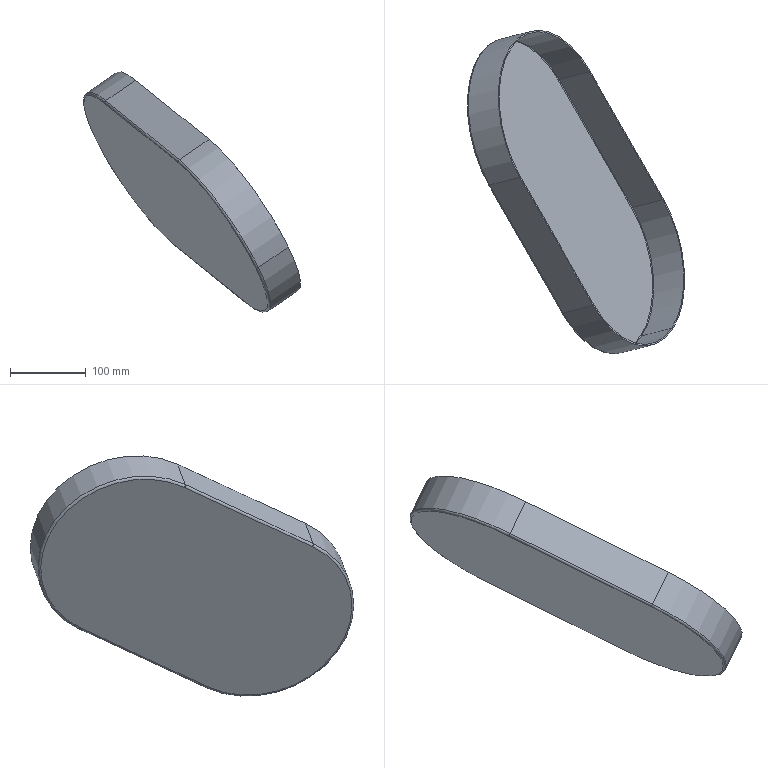Component | SolidWorks | CrusherGearCover-1 | 1 solid | 26 faces | box 287.16 x 427.76 x 317.89 mm | volume 327104 mm3 | cylinder 10 | plane 10 | torus 6 | commonest cylinder face diameters 254 x3 250 x3 2 x2 6 x2
STEP:
#1=COLOUR_RGB('',0.7922,0.8196,0.9333);
#2=FILL_AREA_STYLE_COLOUR('',#1);
#3=FILL_AREA_STYLE('',(#2));
#4=SURFACE_STYLE_FILL_AREA(#3);
#5=SURFACE_SIDE_STYLE('',(#4));
#6=SURFACE_STYLE_USAGE(.BOTH.,#5);
#7=PRESENTATION_STYLE_ASSIGNMENT((#6));
#8=CARTESIAN_POINT('',(-17.886,-16.774,-15.753));
#9=VERTEX_POINT('',#8);
#10=CARTESIAN_POINT('',(-13.854,-17.995,-21.223));
#11=VERTEX_POINT('',#10);
#12=CARTESIAN_POINT('',(-16.107,-14.065,-19.404));
#13=DIRECTION('',(0.8088,0.2094,0.5495));
#14=DIRECTION('',(0.4616,-0.8051,-0.3726));
#15=AXIS2_PLACEMENT_3D('',#12,#13,#14);
#16=CIRCLE('',#15,4.882);
#17=EDGE_CURVE('',#9,#11,#16,.T.);
#18=ORIENTED_EDGE('',*,*,#17,.T.);
#19=CARTESIAN_POINT('',(-13.704,-18.065,-21.202));
#20=VERTEX_POINT('',#19);
#21=CARTESIAN_POINT('',(-13.758,-17.97,-21.158));
#22=DIRECTION('',(-0.3643,-0.555,0.7478));
#23=DIRECTION('',(0.,-0.803,-0.596));
#24=AXIS2_PLACEMENT_3D('',#21,#22,#23);
#25=CIRCLE('',#24,0.1181);
#26=EDGE_CURVE('',#11,#20,#25,.T.);
#27=ORIENTED_EDGE('',*,*,#26,.T.);
#28=CARTESIAN_POINT('',(-17.833,-16.815,-15.6));
#29=VERTEX_POINT('',#28);
#30=CARTESIAN_POINT('',(-16.012,-14.04,-19.339));
#31=DIRECTION('',(0.8088,0.2094,0.5495));
#32=DIRECTION('',(0.4616,-0.8051,-0.3726));
#33=AXIS2_PLACEMENT_3D('',#30,#31,#32);
#34=CIRCLE('',#33,5.);
#35=EDGE_CURVE('',#29,#20,#34,.T.);
#36=ORIENTED_EDGE('',*,*,#35,.F.);
#37=CARTESIAN_POINT('',(-17.79,-16.75,-15.688));
#38=DIRECTION('',(-0.4616,0.8051,0.3726));
#39=DIRECTION('',(-0.3643,-0.555,0.7478));
#40=AXIS2_PLACEMENT_3D('',#37,#38,#39);
#41=CIRCLE('',#40,0.1181);
#42=EDGE_CURVE('',#9,#29,#41,.T.);
#43=ORIENTED_EDGE('',*,*,#42,.F.);
#44=EDGE_LOOP('',(#18,#27,#36,#43));
#45=FACE_OUTER_BOUND('',#44,.T.);
#46=CARTESIAN_POINT('',(-16.012,-14.04,-19.339));
#47=DIRECTION('',(0.8088,0.2094,0.5495));
#48=DIRECTION('',(0.4616,-0.8051,-0.3726));
#49=AXIS2_PLACEMENT_3D('',#46,#47,#48);
#50=TOROIDAL_SURFACE('',#49,4.882,0.1181);
#51=ADVANCED_FACE('',(#45),#50,.T.);
#52=ORIENTED_EDGE('',*,*,#35,.T.);
#53=CARTESIAN_POINT('',(-12.144,-17.661,-20.142));
#54=VERTEX_POINT('',#53);
#55=CARTESIAN_POINT('',(-13.736,-18.074,-21.224));
#56=DIRECTION('',(0.8088,0.2094,0.5495));
#57=VECTOR('',#56,39.37);
#58=LINE('',#55,#57);
#59=EDGE_CURVE('',#20,#54,#58,.T.);
#60=ORIENTED_EDGE('',*,*,#59,.T.);
#61=CARTESIAN_POINT('',(-16.273,-16.411,-14.54));
#62=VERTEX_POINT('',#61);
#63=CARTESIAN_POINT('',(-14.451,-13.636,-18.279));
#64=DIRECTION('',(0.8088,0.2094,0.5495));
#65=DIRECTION('',(0.4616,-0.8051,-0.3726));
#66=AXIS2_PLACEMENT_3D('',#63,#64,#65);
#67=CIRCLE('',#66,5.);
#68=EDGE_CURVE('',#62,#54,#67,.T.);
#69=ORIENTED_EDGE('',*,*,#68,.F.);
#70=CARTESIAN_POINT('',(-17.865,-16.824,-15.621));
#71=DIRECTION('',(0.8088,0.2094,0.5495));
#72=VECTOR('',#71,39.37);
#73=LINE('',#70,#72);
#74=EDGE_CURVE('',#29,#62,#73,.T.);
#75=ORIENTED_EDGE('',*,*,#74,.F.);
#76=EDGE_LOOP('',(#52,#60,#69,#75));
#77=FACE_OUTER_BOUND('',#76,.T.);
#78=CARTESIAN_POINT('',(-16.044,-14.048,-19.361));
#79=DIRECTION('',(0.8088,0.2094,0.5495));
#80=DIRECTION('',(0.4616,-0.8051,-0.3726));
#81=AXIS2_PLACEMENT_3D('',#78,#79,#80);
#82=CYLINDRICAL_SURFACE('',#81,5.);
#83=ADVANCED_FACE('',(#77),#82,.T.);
#84=CARTESIAN_POINT('',(-13.79,-17.979,-21.18));
#85=VERTEX_POINT('',#84);
#86=CARTESIAN_POINT('',(-14.265,-11.339,-23.011));
#87=VERTEX_POINT('',#86);
#88=CARTESIAN_POINT('',(-16.044,-14.048,-19.361));
#89=DIRECTION('',(0.8088,0.2094,0.5495));
#90=DIRECTION('',(-0.3643,-0.555,0.7478));
#91=AXIS2_PLACEMENT_3D('',#88,#89,#90);
#92=CIRCLE('',#91,4.882);
#93=EDGE_CURVE('',#85,#87,#92,.T.);
#94=ORIENTED_EDGE('',*,*,#93,.F.);
#95=CARTESIAN_POINT('',(-13.74,-18.002,-21.173));
#96=VERTEX_POINT('',#95);
#97=CARTESIAN_POINT('',(-13.758,-17.97,-21.158));
#98=DIRECTION('',(-0.3643,-0.555,0.7478));
#99=DIRECTION('',(0.,-0.803,-0.596));
#100=AXIS2_PLACEMENT_3D('',#97,#98,#99);
#101=CIRCLE('',#100,0.03937);
#102=EDGE_CURVE('',#85,#96,#101,.T.);
#103=ORIENTED_EDGE('',*,*,#102,.T.);
#104=CARTESIAN_POINT('',(-14.219,-11.309,-23.019));
#105=VERTEX_POINT('',#104);
#106=CARTESIAN_POINT('',(-16.012,-14.04,-19.339));
#107=DIRECTION('',(0.8088,0.2094,0.5495));
#108=DIRECTION('',(-0.3643,-0.555,0.7478));
#109=AXIS2_PLACEMENT_3D('',#106,#107,#108);
#110=CIRCLE('',#109,4.921);
#111=EDGE_CURVE('',#96,#105,#110,.T.);
#112=ORIENTED_EDGE('',*,*,#111,.T.);
#113=CARTESIAN_POINT('',(-14.233,-11.331,-22.99));
#114=DIRECTION('',(0.4616,-0.8051,-0.3726));
#115=DIRECTION('',(0.8088,0.2094,0.5495));
#116=AXIS2_PLACEMENT_3D('',#113,#114,#115);
#117=CIRCLE('',#116,0.03937);
#118=EDGE_CURVE('',#87,#105,#117,.T.);
#119=ORIENTED_EDGE('',*,*,#118,.F.);
#120=EDGE_LOOP('',(#94,#103,#112,#119));
#121=FACE_OUTER_BOUND('',#120,.T.);
#122=CARTESIAN_POINT('',(-16.012,-14.04,-19.339));
#123=DIRECTION('',(0.8088,0.2094,0.5495));
#124=DIRECTION('',(0.4616,-0.8051,-0.3726));
#125=AXIS2_PLACEMENT_3D('',#122,#123,#124);
#126=TOROIDAL_SURFACE('',#125,4.882,0.03937);
#127=ADVANCED_FACE('',(#121),#126,.F.);
#128=ORIENTED_EDGE('',*,*,#111,.F.);
#129=CARTESIAN_POINT('',(-12.18,-17.598,-20.113));
#130=VERTEX_POINT('',#129);
#131=CARTESIAN_POINT('',(-13.772,-18.01,-21.194));
#132=DIRECTION('',(0.8088,0.2094,0.5495));
#133=VECTOR('',#132,39.37);
#134=LINE('',#131,#133);
#135=EDGE_CURVE('',#96,#130,#134,.T.);
#136=ORIENTED_EDGE('',*,*,#135,.T.);
#137=CARTESIAN_POINT('',(-12.658,-10.905,-21.959));
#138=VERTEX_POINT('',#137);
#139=CARTESIAN_POINT('',(-14.451,-13.636,-18.279));
#140=DIRECTION('',(0.8088,0.2094,0.5495));
#141=DIRECTION('',(-0.3643,-0.555,0.7478));
#142=AXIS2_PLACEMENT_3D('',#139,#140,#141);
#143=CIRCLE('',#142,4.921);
#144=EDGE_CURVE('',#130,#138,#143,.T.);
#145=ORIENTED_EDGE('',*,*,#144,.T.);
#146=CARTESIAN_POINT('',(-14.251,-11.317,-23.041));
#147=DIRECTION('',(0.8088,0.2094,0.5495));
#148=VECTOR('',#147,39.37);
#149=LINE('',#146,#148);
#150=EDGE_CURVE('',#105,#138,#149,.T.);
#151=ORIENTED_EDGE('',*,*,#150,.F.);
#152=EDGE_LOOP('',(#128,#136,#145,#151));
#153=FACE_OUTER_BOUND('',#152,.T.);
#154=CARTESIAN_POINT('',(-16.044,-14.048,-19.361));
#155=DIRECTION('',(0.8088,0.2094,0.5495));
#156=DIRECTION('',(0.4616,-0.8051,-0.3726));
#157=AXIS2_PLACEMENT_3D('',#154,#155,#156);
#158=CYLINDRICAL_SURFACE('',#157,4.921);
#159=ADVANCED_FACE('',(#153),#158,.F.);
#160=CARTESIAN_POINT('',(-16.446,-4.205,-18.937));
#161=VERTEX_POINT('',#160);
#162=CARTESIAN_POINT('',(-16.475,-4.249,-18.878));
#163=VERTEX_POINT('',#162);
#164=CARTESIAN_POINT('',(-16.475,-4.249,-18.878));
#165=DIRECTION('',(-0.3643,-0.555,0.7478));
#166=VECTOR('',#165,39.37);
#167=LINE('',#164,#166);
#168=EDGE_CURVE('',#161,#163,#167,.T.);
#169=ORIENTED_EDGE('',*,*,#168,.F.);
#170=CARTESIAN_POINT('',(-20.089,-9.755,-11.459));
#171=VERTEX_POINT('',#170);
#172=CARTESIAN_POINT('',(-18.268,-6.98,-15.198));
#173=DIRECTION('',(0.8088,0.2094,0.5495));
#174=DIRECTION('',(0.4616,-0.8051,-0.3726));
#175=AXIS2_PLACEMENT_3D('',#172,#173,#174);
#176=CIRCLE('',#175,5.);
#177=EDGE_CURVE('',#161,#171,#176,.T.);
#178=ORIENTED_EDGE('',*,*,#177,.T.);
#179=CARTESIAN_POINT('',(-20.061,-9.712,-11.518));
#180=VERTEX_POINT('',#179);
#181=CARTESIAN_POINT('',(-20.061,-9.712,-11.518));
#182=DIRECTION('',(0.3643,0.555,-0.7478));
#183=VECTOR('',#182,39.37);
#184=LINE('',#181,#183);
#185=EDGE_CURVE('',#171,#180,#184,.T.);
#186=ORIENTED_EDGE('',*,*,#185,.T.);
#187=CARTESIAN_POINT('',(-18.268,-6.98,-15.198));
#188=DIRECTION('',(0.8088,0.2094,0.5495));
#189=DIRECTION('',(0.3643,0.555,-0.7478));
#190=AXIS2_PLACEMENT_3D('',#187,#188,#189);
#191=CIRCLE('',#190,4.921);
#192=EDGE_CURVE('',#163,#180,#191,.T.);
#193=ORIENTED_EDGE('',*,*,#192,.F.);
#194=EDGE_LOOP('',(#169,#178,#186,#193));
#195=FACE_OUTER_BOUND('',#194,.T.);
#196=CARTESIAN_POINT('',(-18.268,-6.98,-15.198));
#197=DIRECTION('',(-0.8088,-0.2094,-0.5495));
#198=DIRECTION('',(-0.4616,0.8051,0.3726));
#199=AXIS2_PLACEMENT_3D('',#196,#197,#198);
#200=PLANE('',#199);
#201=ADVANCED_FACE('',(#195),#200,.F.);
#202=ORIENTED_EDGE('',*,*,#185,.F.);
#203=CARTESIAN_POINT('',(-20.089,-9.755,-11.459));
#204=DIRECTION('',(0.4616,-0.8051,-0.3726));
#205=VECTOR('',#204,39.37);
#206=LINE('',#203,#205);
#207=EDGE_CURVE('',#171,#62,#206,.T.);
#208=ORIENTED_EDGE('',*,*,#207,.T.);
#209=CARTESIAN_POINT('',(-16.244,-16.368,-14.599));
#210=VERTEX_POINT('',#209);
#211=CARTESIAN_POINT('',(-16.244,-16.368,-14.599));
#212=DIRECTION('',(0.3643,0.555,-0.7478));
#213=VECTOR('',#212,39.37);
#214=LINE('',#211,#213);
#215=EDGE_CURVE('',#62,#210,#214,.T.);
#216=ORIENTED_EDGE('',*,*,#215,.T.);
#217=CARTESIAN_POINT('',(-20.061,-9.712,-11.518));
#218=DIRECTION('',(0.4616,-0.8051,-0.3726));
#219=VECTOR('',#218,39.37);
#220=LINE('',#217,#219);
#221=EDGE_CURVE('',#180,#210,#220,.T.);
#222=ORIENTED_EDGE('',*,*,#221,.F.);
#223=EDGE_LOOP('',(#202,#208,#216,#222));
#224=FACE_OUTER_BOUND('',#223,.T.);
#225=CARTESIAN_POINT('',(-20.061,-9.712,-11.518));
#226=DIRECTION('',(0.8088,0.2094,0.5495));
#227=DIRECTION('',(0.4616,-0.8051,-0.3726));
#228=AXIS2_PLACEMENT_3D('',#225,#226,#227);
#229=PLANE('',#228);
#230=ADVANCED_FACE('',(#224),#229,.T.);
#231=ORIENTED_EDGE('',*,*,#215,.F.);
#232=ORIENTED_EDGE('',*,*,#68,.T.);
#233=CARTESIAN_POINT('',(-12.63,-10.861,-22.018));
#234=VERTEX_POINT('',#233);
#235=CARTESIAN_POINT('',(-14.451,-13.636,-18.279));
#236=DIRECTION('',(0.8088,0.2094,0.5495));
#237=DIRECTION('',(0.4616,-0.8051,-0.3726));
#238=AXIS2_PLACEMENT_3D('',#235,#236,#237);
#239=CIRCLE('',#238,5.);
#240=EDGE_CURVE('',#54,#234,#239,.T.);
#241=ORIENTED_EDGE('',*,*,#240,.T.);
#242=CARTESIAN_POINT('',(-12.658,-10.905,-21.959));
#243=DIRECTION('',(-0.3643,-0.555,0.7478));
#244=VECTOR('',#243,39.37);
#245=LINE('',#242,#244);
#246=EDGE_CURVE('',#234,#138,#245,.T.);
#247=ORIENTED_EDGE('',*,*,#246,.T.);
#248=ORIENTED_EDGE('',*,*,#144,.F.);
#249=CARTESIAN_POINT('',(-14.451,-13.636,-18.279));
#250=DIRECTION('',(0.8088,0.2094,0.5495));
#251=DIRECTION('',(-0.3643,-0.555,0.7478));
#252=AXIS2_PLACEMENT_3D('',#249,#250,#251);
#253=CIRCLE('',#252,4.921);
#254=EDGE_CURVE('',#210,#130,#253,.T.);
#255=ORIENTED_EDGE('',*,*,#254,.F.);
#256=EDGE_LOOP('',(#231,#232,#241,#247,#248,#255));
#257=FACE_OUTER_BOUND('',#256,.T.);
#258=CARTESIAN_POINT('',(-14.451,-13.636,-18.279));
#259=DIRECTION('',(-0.8088,-0.2094,-0.5495));
#260=DIRECTION('',(-0.4616,0.8051,0.3726));
#261=AXIS2_PLACEMENT_3D('',#258,#259,#260);
#262=PLANE('',#261);
#263=ADVANCED_FACE('',(#257),#262,.F.);
#264=CARTESIAN_POINT('',(-12.63,-10.861,-22.018));
#265=DIRECTION('',(-0.4616,0.8051,0.3726));
#266=VECTOR('',#265,39.37);
#267=LINE('',#264,#266);
#268=EDGE_CURVE('',#234,#161,#267,.T.);
#269=ORIENTED_EDGE('',*,*,#268,.T.);
#270=ORIENTED_EDGE('',*,*,#168,.T.);
#271=CARTESIAN_POINT('',(-12.658,-10.905,-21.959));
#272=DIRECTION('',(-0.4616,0.8051,0.3726));
#273=VECTOR('',#272,39.37);
#274=LINE('',#271,#273);
#275=EDGE_CURVE('',#138,#163,#274,.T.);
#276=ORIENTED_EDGE('',*,*,#275,.F.);
#277=ORIENTED_EDGE('',*,*,#246,.F.);
#278=EDGE_LOOP('',(#269,#270,#276,#277));
#279=FACE_OUTER_BOUND('',#278,.T.);
#280=CARTESIAN_POINT('',(-12.658,-10.905,-21.959));
#281=DIRECTION('',(0.8088,0.2094,0.5495));
#282=DIRECTION('',(-0.4616,0.8051,0.3726));
#283=AXIS2_PLACEMENT_3D('',#280,#281,#282);
#284=PLANE('',#283);
#285=ADVANCED_FACE('',(#279),#284,.T.);
#286=ORIENTED_EDGE('',*,*,#135,.F.);
#287=CARTESIAN_POINT('',(-17.805,-16.772,-15.659));
#288=VERTEX_POINT('',#287);
#289=CARTESIAN_POINT('',(-16.012,-14.04,-19.339));
#290=DIRECTION('',(0.8088,0.2094,0.5495));
#291=DIRECTION('',(-0.3643,-0.555,0.7478));
#292=AXIS2_PLACEMENT_3D('',#289,#290,#291);
#293=CIRCLE('',#292,4.921);
#294=EDGE_CURVE('',#288,#96,#293,.T.);
#295=ORIENTED_EDGE('',*,*,#294,.F.);
#296=CARTESIAN_POINT('',(-17.837,-16.78,-15.68));
#297=DIRECTION('',(0.8088,0.2094,0.5495));
#298=VECTOR('',#297,39.37);
#299=LINE('',#296,#298);
#300=EDGE_CURVE('',#288,#210,#299,.T.);
#301=ORIENTED_EDGE('',*,*,#300,.T.);
#302=ORIENTED_EDGE('',*,*,#254,.T.);
#303=EDGE_LOOP('',(#286,#295,#301,#302));
#304=FACE_OUTER_BOUND('',#303,.T.);
#305=CARTESIAN_POINT('',(-16.044,-14.048,-19.361));
#306=DIRECTION('',(0.8088,0.2094,0.5495));
#307=DIRECTION('',(0.4616,-0.8051,-0.3726));
#308=AXIS2_PLACEMENT_3D('',#305,#306,#307);
#309=CYLINDRICAL_SURFACE('',#308,4.921);
#310=ADVANCED_FACE('',(#304),#309,.F.);
#311=ORIENTED_EDGE('',*,*,#102,.F.);
#312=CARTESIAN_POINT('',(-17.822,-16.758,-15.71));
#313=VERTEX_POINT('',#312);
#314=CARTESIAN_POINT('',(-16.044,-14.048,-19.361));
#315=DIRECTION('',(0.8088,0.2094,0.5495));
#316=DIRECTION('',(-0.3643,-0.555,0.7478));
#317=AXIS2_PLACEMENT_3D('',#314,#315,#316);
#318=CIRCLE('',#317,4.882);
#319=EDGE_CURVE('',#313,#85,#318,.T.);
#320=ORIENTED_EDGE('',*,*,#319,.F.);
#321=CARTESIAN_POINT('',(-17.79,-16.75,-15.688));
#322=DIRECTION('',(-0.4616,0.8051,0.3726));
#323=DIRECTION('',(0.8088,0.2094,0.5495));
#324=AXIS2_PLACEMENT_3D('',#321,#322,#323);
#325=CIRCLE('',#324,0.03937);
#326=EDGE_CURVE('',#313,#288,#325,.T.);
#327=ORIENTED_EDGE('',*,*,#326,.T.);
#328=ORIENTED_EDGE('',*,*,#294,.T.);
#329=EDGE_LOOP('',(#311,#320,#327,#328));
#330=FACE_OUTER_BOUND('',#329,.T.);
#331=CARTESIAN_POINT('',(-16.012,-14.04,-19.339));
#332=DIRECTION('',(0.8088,0.2094,0.5495));
#333=DIRECTION('',(0.4616,-0.8051,-0.3726));
#334=AXIS2_PLACEMENT_3D('',#331,#332,#333);
#335=TOROIDAL_SURFACE('',#334,4.882,0.03937);
#336=ADVANCED_FACE('',(#330),#335,.F.);
#337=ORIENTED_EDGE('',*,*,#221,.T.);
#338=ORIENTED_EDGE('',*,*,#300,.F.);
#339=CARTESIAN_POINT('',(-21.621,-10.116,-12.578));
#340=VERTEX_POINT('',#339);
#341=CARTESIAN_POINT('',(-21.621,-10.116,-12.578));
#342=DIRECTION('',(0.4616,-0.8051,-0.3726));
#343=VECTOR('',#342,39.37);
#344=LINE('',#341,#343);
#345=EDGE_CURVE('',#340,#288,#344,.T.);
#346=ORIENTED_EDGE('',*,*,#345,.F.);
#347=CARTESIAN_POINT('',(-21.653,-10.124,-12.6));
#348=DIRECTION('',(0.8088,0.2094,0.5495));
#349=VECTOR('',#348,39.37);
#350=LINE('',#347,#349);
#351=EDGE_CURVE('',#340,#180,#350,.T.);
#352=ORIENTED_EDGE('',*,*,#351,.T.);
#353=EDGE_LOOP('',(#337,#338,#346,#352));
#354=FACE_OUTER_BOUND('',#353,.T.);
#355=CARTESIAN_POINT('',(-21.653,-10.124,-12.6));
#356=DIRECTION('',(0.3643,0.555,-0.7478));
#357=DIRECTION('',(0.8088,0.2094,0.5495));
#358=AXIS2_PLACEMENT_3D('',#355,#356,#357);
#359=PLANE('',#358);
#360=ADVANCED_FACE('',(#354),#359,.T.);
#361=ORIENTED_EDGE('',*,*,#345,.T.);
#362=ORIENTED_EDGE('',*,*,#326,.F.);
#363=CARTESIAN_POINT('',(-21.638,-10.102,-12.629));
#364=VERTEX_POINT('',#363);
#365=CARTESIAN_POINT('',(-21.638,-10.102,-12.629));
#366=DIRECTION('',(0.4616,-0.8051,-0.3726));
#367=VECTOR('',#366,39.37);
#368=LINE('',#365,#367);
#369=EDGE_CURVE('',#364,#313,#368,.T.);
#370=ORIENTED_EDGE('',*,*,#369,.F.);
#371=CARTESIAN_POINT('',(-21.607,-10.094,-12.607));
#372=DIRECTION('',(-0.4616,0.8051,0.3726));
#373=DIRECTION('',(0.8088,0.2094,0.5495));
#374=AXIS2_PLACEMENT_3D('',#371,#372,#373);
#375=CIRCLE('',#374,0.03937);
#376=EDGE_CURVE('',#364,#340,#375,.T.);
#377=ORIENTED_EDGE('',*,*,#376,.T.);
#378=EDGE_LOOP('',(#361,#362,#370,#377));
#379=FACE_OUTER_BOUND('',#378,.T.);
#380=CARTESIAN_POINT('',(-21.607,-10.094,-12.607));
#381=DIRECTION('',(0.4616,-0.8051,-0.3726));
#382=DIRECTION('',(-0.8088,-0.2094,-0.5495));
#383=AXIS2_PLACEMENT_3D('',#380,#381,#382);
#384=CYLINDRICAL_SURFACE('',#383,0.03937);
#385=ADVANCED_FACE('',(#379),#384,.F.);
#386=ORIENTED_EDGE('',*,*,#192,.T.);
#387=ORIENTED_EDGE('',*,*,#351,.F.);
#388=CARTESIAN_POINT('',(-18.035,-4.653,-19.938));
#389=VERTEX_POINT('',#388);
#390=CARTESIAN_POINT('',(-19.828,-7.384,-16.258));
#391=DIRECTION('',(0.8088,0.2094,0.5495));
#392=DIRECTION('',(0.3643,0.555,-0.7478));
#393=AXIS2_PLACEMENT_3D('',#390,#391,#392);
#394=CIRCLE('',#393,4.921);
#395=EDGE_CURVE('',#389,#340,#394,.T.);
#396=ORIENTED_EDGE('',*,*,#395,.F.);
#397=CARTESIAN_POINT('',(-18.067,-4.661,-19.96));
#398=DIRECTION('',(0.8088,0.2094,0.5495));
#399=VECTOR('',#398,39.37);
#400=LINE('',#397,#399);
#401=EDGE_CURVE('',#389,#163,#400,.T.);
#402=ORIENTED_EDGE('',*,*,#401,.T.);
#403=EDGE_LOOP('',(#386,#387,#396,#402));
#404=FACE_OUTER_BOUND('',#403,.T.);
#405=CARTESIAN_POINT('',(-19.86,-7.393,-16.28));
#406=DIRECTION('',(0.8088,0.2094,0.5495));
#407=DIRECTION('',(0.4616,-0.8051,-0.3726));
#408=AXIS2_PLACEMENT_3D('',#405,#406,#407);
#409=CYLINDRICAL_SURFACE('',#408,4.921);
#410=ADVANCED_FACE('',(#404),#409,.F.);
#411=ORIENTED_EDGE('',*,*,#395,.T.);
#412=ORIENTED_EDGE('',*,*,#376,.F.);
#413=CARTESIAN_POINT('',(-18.081,-4.683,-19.931));
#414=VERTEX_POINT('',#413);
#415=CARTESIAN_POINT('',(-19.86,-7.393,-16.28));
#416=DIRECTION('',(0.8088,0.2094,0.5495));
#417=DIRECTION('',(0.3643,0.555,-0.7478));
#418=AXIS2_PLACEMENT_3D('',#415,#416,#417);
#419=CIRCLE('',#418,4.882);
#420=EDGE_CURVE('',#414,#364,#419,.T.);
#421=ORIENTED_EDGE('',*,*,#420,.F.);
#422=CARTESIAN_POINT('',(-18.049,-4.675,-19.909));
#423=DIRECTION('',(0.4616,-0.8051,-0.3726));
#424=DIRECTION('',(0.8088,0.2094,0.5495));
#425=AXIS2_PLACEMENT_3D('',#422,#423,#424);
#426=CIRCLE('',#425,0.03937);
#427=EDGE_CURVE('',#414,#389,#426,.T.);
#428=ORIENTED_EDGE('',*,*,#427,.T.);
#429=EDGE_LOOP('',(#411,#412,#421,#428));
#430=FACE_OUTER_BOUND('',#429,.T.);
#431=CARTESIAN_POINT('',(-19.828,-7.384,-16.258));
#432=DIRECTION('',(0.8088,0.2094,0.5495));
#433=DIRECTION('',(0.4616,-0.8051,-0.3726));
#434=AXIS2_PLACEMENT_3D('',#431,#432,#433);
#435=TOROIDAL_SURFACE('',#434,4.882,0.03937);
#436=ADVANCED_FACE('',(#430),#435,.F.);
#437=ORIENTED_EDGE('',*,*,#275,.T.);
#438=ORIENTED_EDGE('',*,*,#401,.F.);
#439=CARTESIAN_POINT('',(-14.219,-11.309,-23.019));
#440=DIRECTION('',(-0.4616,0.8051,0.3726));
#441=VECTOR('',#440,39.37);
#442=LINE('',#439,#441);
#443=EDGE_CURVE('',#105,#389,#442,.T.);
#444=ORIENTED_EDGE('',*,*,#443,.F.);
#445=ORIENTED_EDGE('',*,*,#150,.T.);
#446=EDGE_LOOP('',(#437,#438,#444,#445));
#447=FACE_OUTER_BOUND('',#446,.T.);
#448=CARTESIAN_POINT('',(-14.251,-11.317,-23.041));
#449=DIRECTION('',(-0.3643,-0.555,0.7478));
#450=DIRECTION('',(-0.8088,-0.2094,-0.5495));
#451=AXIS2_PLACEMENT_3D('',#448,#449,#450);
#452=PLANE('',#451);
#453=ADVANCED_FACE('',(#447),#452,.T.);
#454=ORIENTED_EDGE('',*,*,#443,.T.);
#455=ORIENTED_EDGE('',*,*,#427,.F.);
#456=CARTESIAN_POINT('',(-14.265,-11.339,-23.011));
#457=DIRECTION('',(-0.4616,0.8051,0.3726));
#458=VECTOR('',#457,39.37);
#459=LINE('',#456,#458);
#460=EDGE_CURVE('',#87,#414,#459,.T.);
#461=ORIENTED_EDGE('',*,*,#460,.F.);
#462=ORIENTED_EDGE('',*,*,#118,.T.);
#463=EDGE_LOOP('',(#454,#455,#461,#462));
#464=FACE_OUTER_BOUND('',#463,.T.);
#465=CARTESIAN_POINT('',(-14.233,-11.331,-22.99));
#466=DIRECTION('',(-0.4616,0.8051,0.3726));
#467=DIRECTION('',(0.8088,0.2094,0.5495));
#468=AXIS2_PLACEMENT_3D('',#465,#466,#467);
#469=CYLINDRICAL_SURFACE('',#468,0.03937);
#470=ADVANCED_FACE('',(#464),#469,.F.);
#471=ORIENTED_EDGE('',*,*,#59,.F.);
#472=CARTESIAN_POINT('',(-14.19,-11.265,-23.078));
#473=VERTEX_POINT('',#472);
#474=CARTESIAN_POINT('',(-16.012,-14.04,-19.339));
#475=DIRECTION('',(0.8088,0.2094,0.5495));
#476=DIRECTION('',(0.4616,-0.8051,-0.3726));
#477=AXIS2_PLACEMENT_3D('',#474,#475,#476);
#478=CIRCLE('',#477,5.);
#479=EDGE_CURVE('',#20,#473,#478,.T.);
#480=ORIENTED_EDGE('',*,*,#479,.T.);
#481=CARTESIAN_POINT('',(-14.222,-11.273,-23.1));
#482=DIRECTION('',(0.8088,0.2094,0.5495));
#483=VECTOR('',#482,39.37);
#484=LINE('',#481,#483);
#485=EDGE_CURVE('',#473,#234,#484,.T.);
#486=ORIENTED_EDGE('',*,*,#485,.T.);
#487=ORIENTED_EDGE('',*,*,#240,.F.);
#488=EDGE_LOOP('',(#471,#480,#486,#487));
#489=FACE_OUTER_BOUND('',#488,.T.);
#490=CARTESIAN_POINT('',(-16.044,-14.048,-19.361));
#491=DIRECTION('',(0.8088,0.2094,0.5495));
#492=DIRECTION('',(0.4616,-0.8051,-0.3726));
#493=AXIS2_PLACEMENT_3D('',#490,#491,#492);
#494=CYLINDRICAL_SURFACE('',#493,5.);
#495=ADVANCED_FACE('',(#489),#494,.T.);
#496=ORIENTED_EDGE('',*,*,#26,.F.);
#497=CARTESIAN_POINT('',(-14.329,-11.355,-23.055));
#498=VERTEX_POINT('',#497);
#499=CARTESIAN_POINT('',(-16.107,-14.065,-19.404));
#500=DIRECTION('',(0.8088,0.2094,0.5495));
#501=DIRECTION('',(0.4616,-0.8051,-0.3726));
#502=AXIS2_PLACEMENT_3D('',#499,#500,#501);
#503=CIRCLE('',#502,4.882);
#504=EDGE_CURVE('',#11,#498,#503,.T.);
#505=ORIENTED_EDGE('',*,*,#504,.T.);
#506=CARTESIAN_POINT('',(-14.233,-11.331,-22.99));
#507=DIRECTION('',(0.4616,-0.8051,-0.3726));
#508=DIRECTION('',(0.8088,0.2094,0.5495));
#509=AXIS2_PLACEMENT_3D('',#506,#507,#508);
#510=CIRCLE('',#509,0.1181);
#511=EDGE_CURVE('',#498,#473,#510,.T.);
#512=ORIENTED_EDGE('',*,*,#511,.T.);
#513=ORIENTED_EDGE('',*,*,#479,.F.);
#514=EDGE_LOOP('',(#496,#505,#512,#513));
#515=FACE_OUTER_BOUND('',#514,.T.);
#516=CARTESIAN_POINT('',(-16.012,-14.04,-19.339));
#517=DIRECTION('',(0.8088,0.2094,0.5495));
#518=DIRECTION('',(0.4616,-0.8051,-0.3726));
#519=AXIS2_PLACEMENT_3D('',#516,#517,#518);
#520=TOROIDAL_SURFACE('',#519,4.882,0.1181);
#521=ADVANCED_FACE('',(#515),#520,.T.);
#522=ORIENTED_EDGE('',*,*,#207,.F.);
#523=CARTESIAN_POINT('',(-21.65,-10.159,-12.519));
#524=VERTEX_POINT('',#523);
#525=CARTESIAN_POINT('',(-21.681,-10.168,-12.541));
#526=DIRECTION('',(0.8088,0.2094,0.5495));
#527=VECTOR('',#526,39.37);
#528=LINE('',#525,#527);
#529=EDGE_CURVE('',#524,#171,#528,.T.);
#530=ORIENTED_EDGE('',*,*,#529,.F.);
#531=CARTESIAN_POINT('',(-21.65,-10.159,-12.519));
#532=DIRECTION('',(0.4616,-0.8051,-0.3726));
#533=VECTOR('',#532,39.37);
#534=LINE('',#531,#533);
#535=EDGE_CURVE('',#524,#29,#534,.T.);
#536=ORIENTED_EDGE('',*,*,#535,.T.);
#537=ORIENTED_EDGE('',*,*,#74,.T.);
#538=EDGE_LOOP('',(#522,#530,#536,#537));
#539=FACE_OUTER_BOUND('',#538,.T.);
#540=CARTESIAN_POINT('',(-21.681,-10.168,-12.541));
#541=DIRECTION('',(0.3643,0.555,-0.7478));
#542=DIRECTION('',(0.8088,0.2094,0.5495));
#543=AXIS2_PLACEMENT_3D('',#540,#541,#542);
#544=PLANE('',#543);
#545=ADVANCED_FACE('',(#539),#544,.F.);
#546=ORIENTED_EDGE('',*,*,#535,.F.);
#547=CARTESIAN_POINT('',(-21.702,-10.119,-12.672));
#548=VERTEX_POINT('',#547);
#549=CARTESIAN_POINT('',(-21.607,-10.094,-12.607));
#550=DIRECTION('',(-0.4616,0.8051,0.3726));
#551=DIRECTION('',(-0.8088,-0.2094,-0.5495));
#552=AXIS2_PLACEMENT_3D('',#549,#550,#551);
#553=CIRCLE('',#552,0.1181);
#554=EDGE_CURVE('',#548,#524,#553,.T.);
#555=ORIENTED_EDGE('',*,*,#554,.F.);
#556=CARTESIAN_POINT('',(-19.794,-13.447,-14.213));
#557=DIRECTION('',(0.4616,-0.8051,-0.3726));
#558=VECTOR('',#557,39.37);
#559=LINE('',#556,#558);
#560=EDGE_CURVE('',#548,#9,#559,.T.);
#561=ORIENTED_EDGE('',*,*,#560,.T.);
#562=ORIENTED_EDGE('',*,*,#42,.T.);
#563=EDGE_LOOP('',(#546,#555,#561,#562));
#564=FACE_OUTER_BOUND('',#563,.T.);
#565=CARTESIAN_POINT('',(-21.607,-10.094,-12.607));
#566=DIRECTION('',(0.4616,-0.8051,-0.3726));
#567=DIRECTION('',(-0.8088,-0.2094,-0.5495));
#568=AXIS2_PLACEMENT_3D('',#565,#566,#567);
#569=CYLINDRICAL_SURFACE('',#568,0.1181);
#570=ADVANCED_FACE('',(#564),#569,.T.);
#571=ORIENTED_EDGE('',*,*,#177,.F.);
#572=CARTESIAN_POINT('',(-18.006,-4.609,-19.997));
#573=VERTEX_POINT('',#572);
#574=CARTESIAN_POINT('',(-18.038,-4.617,-20.019));
#575=DIRECTION('',(0.8088,0.2094,0.5495));
#576=VECTOR('',#575,39.37);
#577=LINE('',#574,#576);
#578=EDGE_CURVE('',#573,#161,#577,.T.);
#579=ORIENTED_EDGE('',*,*,#578,.F.);
#580=CARTESIAN_POINT('',(-19.828,-7.384,-16.258));
#581=DIRECTION('',(0.8088,0.2094,0.5495));
#582=DIRECTION('',(0.4616,-0.8051,-0.3726));
#583=AXIS2_PLACEMENT_3D('',#580,#581,#582);
#584=CIRCLE('',#583,5.);
#585=EDGE_CURVE('',#573,#524,#584,.T.);
#586=ORIENTED_EDGE('',*,*,#585,.T.);
#587=ORIENTED_EDGE('',*,*,#529,.T.);
#588=EDGE_LOOP('',(#571,#579,#586,#587));
#589=FACE_OUTER_BOUND('',#588,.T.);
#590=CARTESIAN_POINT('',(-19.86,-7.393,-16.28));
#591=DIRECTION('',(0.8088,0.2094,0.5495));
#592=DIRECTION('',(0.4616,-0.8051,-0.3726));
#593=AXIS2_PLACEMENT_3D('',#590,#591,#592);
#594=CYLINDRICAL_SURFACE('',#593,5.);
#595=ADVANCED_FACE('',(#589),#594,.T.);
#596=ORIENTED_EDGE('',*,*,#585,.F.);
#597=CARTESIAN_POINT('',(-18.145,-4.7,-19.974));
#598=VERTEX_POINT('',#597);
#599=CARTESIAN_POINT('',(-18.049,-4.675,-19.909));
#600=DIRECTION('',(0.4616,-0.8051,-0.3726));
#601=DIRECTION('',(0.3643,0.555,-0.7478));
#602=AXIS2_PLACEMENT_3D('',#599,#600,#601);
#603=CIRCLE('',#602,0.1181);
#604=EDGE_CURVE('',#598,#573,#603,.T.);
#605=ORIENTED_EDGE('',*,*,#604,.F.);
#606=CARTESIAN_POINT('',(-19.923,-7.409,-16.323));
#607=DIRECTION('',(0.8088,0.2094,0.5495));
#608=DIRECTION('',(0.4616,-0.8051,-0.3726));
#609=AXIS2_PLACEMENT_3D('',#606,#607,#608);
#610=CIRCLE('',#609,4.882);
#611=EDGE_CURVE('',#598,#548,#610,.T.);
#612=ORIENTED_EDGE('',*,*,#611,.T.);
#613=ORIENTED_EDGE('',*,*,#554,.T.);
#614=EDGE_LOOP('',(#596,#605,#612,#613));
#615=FACE_OUTER_BOUND('',#614,.T.);
#616=CARTESIAN_POINT('',(-19.828,-7.384,-16.258));
#617=DIRECTION('',(0.8088,0.2094,0.5495));
#618=DIRECTION('',(0.4616,-0.8051,-0.3726));
#619=AXIS2_PLACEMENT_3D('',#616,#617,#618);
#620=TOROIDAL_SURFACE('',#619,4.882,0.1181);
#621=ADVANCED_FACE('',(#615),#620,.T.);
#622=ORIENTED_EDGE('',*,*,#268,.F.);
#623=ORIENTED_EDGE('',*,*,#485,.F.);
#624=CARTESIAN_POINT('',(-14.19,-11.265,-23.078));
#625=DIRECTION('',(-0.4616,0.8051,0.3726));
#626=VECTOR('',#625,39.37);
#627=LINE('',#624,#626);
#628=EDGE_CURVE('',#473,#573,#627,.T.);
#629=ORIENTED_EDGE('',*,*,#628,.T.);
#630=ORIENTED_EDGE('',*,*,#578,.T.);
#631=EDGE_LOOP('',(#622,#623,#629,#630));
#632=FACE_OUTER_BOUND('',#631,.T.);
#633=CARTESIAN_POINT('',(-14.222,-11.273,-23.1));
#634=DIRECTION('',(-0.3643,-0.555,0.7478));
#635=DIRECTION('',(-0.8088,-0.2094,-0.5495));
#636=AXIS2_PLACEMENT_3D('',#633,#634,#635);
#637=PLANE('',#636);
#638=ADVANCED_FACE('',(#632),#637,.F.);
#639=ORIENTED_EDGE('',*,*,#628,.F.);
#640=ORIENTED_EDGE('',*,*,#511,.F.);
#641=CARTESIAN_POINT('',(-14.329,-11.355,-23.055));
#642=DIRECTION('',(-0.4616,0.8051,0.3726));
#643=VECTOR('',#642,39.37);
#644=LINE('',#641,#643);
#645=EDGE_CURVE('',#498,#598,#644,.T.);
#646=ORIENTED_EDGE('',*,*,#645,.T.);
#647=ORIENTED_EDGE('',*,*,#604,.T.);
#648=EDGE_LOOP('',(#639,#640,#646,#647));
#649=FACE_OUTER_BOUND('',#648,.T.);
#650=CARTESIAN_POINT('',(-14.233,-11.331,-22.99));
#651=DIRECTION('',(-0.4616,0.8051,0.3726));
#652=DIRECTION('',(0.8088,0.2094,0.5495));
#653=AXIS2_PLACEMENT_3D('',#650,#651,#652);
#654=CYLINDRICAL_SURFACE('',#653,0.1181);
#655=ADVANCED_FACE('',(#649),#654,.T.);
#656=ORIENTED_EDGE('',*,*,#319,.T.);
#657=ORIENTED_EDGE('',*,*,#93,.T.);
#658=ORIENTED_EDGE('',*,*,#460,.T.);
#659=ORIENTED_EDGE('',*,*,#420,.T.);
#660=ORIENTED_EDGE('',*,*,#369,.T.);
#661=EDGE_LOOP('',(#656,#657,#658,#659,#660));
#662=FACE_OUTER_BOUND('',#661,.T.);
#663=CARTESIAN_POINT('',(-19.86,-7.393,-16.28));
#664=DIRECTION('',(0.8088,0.2094,0.5495));
#665=DIRECTION('',(0.4616,-0.8051,-0.3726));
#666=AXIS2_PLACEMENT_3D('',#663,#664,#665);
#667=PLANE('',#666);
#668=ADVANCED_FACE('',(#662),#667,.T.);
#669=ORIENTED_EDGE('',*,*,#645,.F.);
#670=ORIENTED_EDGE('',*,*,#504,.F.);
#671=ORIENTED_EDGE('',*,*,#17,.F.);
#672=ORIENTED_EDGE('',*,*,#560,.F.);
#673=ORIENTED_EDGE('',*,*,#611,.F.);
#674=EDGE_LOOP('',(#669,#670,#671,#672,#673));
#675=FACE_OUTER_BOUND('',#674,.T.);
#676=CARTESIAN_POINT('',(-19.923,-7.409,-16.323));
#677=DIRECTION('',(0.8088,0.2094,0.5495));
#678=DIRECTION('',(0.4616,-0.8051,-0.3726));
#679=AXIS2_PLACEMENT_3D('',#676,#677,#678);
#680=PLANE('',#679);
#681=ADVANCED_FACE('',(#675),#680,.F.);
#682=CLOSED_SHELL('',(#51,#83,#127,#159,#201,#230,#263,#285,#310,#336,#360,#385,#410,#436,#453,#470,#495,#521,#545,#570,#595,#621,#638,#655,#668,#681));
#683=MANIFOLD_SOLID_BREP('',#682);
#684=STYLED_ITEM('',(#7),#683);
#685=(LENGTH_UNIT()NAMED_UNIT(*)SI_UNIT($,.METRE.));
#686=LENGTH_MEASURE_WITH_UNIT(LENGTH_MEASURE(0.0254),#685);
#687=DIMENSIONAL_EXPONENTS(1.,0.,0.,0.,0.,0.,0.);
#688=(CONVERSION_BASED_UNIT('',#686)LENGTH_UNIT()NAMED_UNIT(#687));
#689=UNCERTAINTY_MEASURE_WITH_UNIT(LENGTH_MEASURE(0.00001),#688,'','');
#690=(NAMED_UNIT(*)PLANE_ANGLE_UNIT()SI_UNIT($,.RADIAN.));
#691=(NAMED_UNIT(*)SI_UNIT($,.STERADIAN.)SOLID_ANGLE_UNIT());
#692=(GEOMETRIC_REPRESENTATION_CONTEXT(3)GLOBAL_UNCERTAINTY_ASSIGNED_CONTEXT((#689))GLOBAL_UNIT_ASSIGNED_CONTEXT((#688,#690,#691))REPRESENTATION_CONTEXT('',''));
#693=MECHANICAL_DESIGN_GEOMETRIC_PRESENTATION_REPRESENTATION('',(#684),#692);
#694=CARTESIAN_POINT('',(0.,0.,0.));
#695=DIRECTION('',(0.,0.,1.));
#696=DIRECTION('',(1.,0.,0.));
#697=AXIS2_PLACEMENT_3D('',#694,#695,#696);
#698=(LENGTH_UNIT()NAMED_UNIT(*)SI_UNIT($,.METRE.));
#699=LENGTH_MEASURE_WITH_UNIT(LENGTH_MEASURE(0.0254),#698);
#700=DIMENSIONAL_EXPONENTS(1.,0.,0.,0.,0.,0.,0.);
#701=(CONVERSION_BASED_UNIT('',#699)LENGTH_UNIT()NAMED_UNIT(#700));
#702=UNCERTAINTY_MEASURE_WITH_UNIT(LENGTH_MEASURE(0.00001),#701,'','');
#703=(NAMED_UNIT(*)PLANE_ANGLE_UNIT()SI_UNIT($,.RADIAN.));
#704=(NAMED_UNIT(*)SI_UNIT($,.STERADIAN.)SOLID_ANGLE_UNIT());
#705=(GEOMETRIC_REPRESENTATION_CONTEXT(3)GLOBAL_UNCERTAINTY_ASSIGNED_CONTEXT((#702))GLOBAL_UNIT_ASSIGNED_CONTEXT((#701,#703,#704))REPRESENTATION_CONTEXT('',''));
#706=ADVANCED_BREP_SHAPE_REPRESENTATION('',(#683,#697),#705);
#707=PRESENTATION_LAYER_ASSIGNMENT('','',(#684));